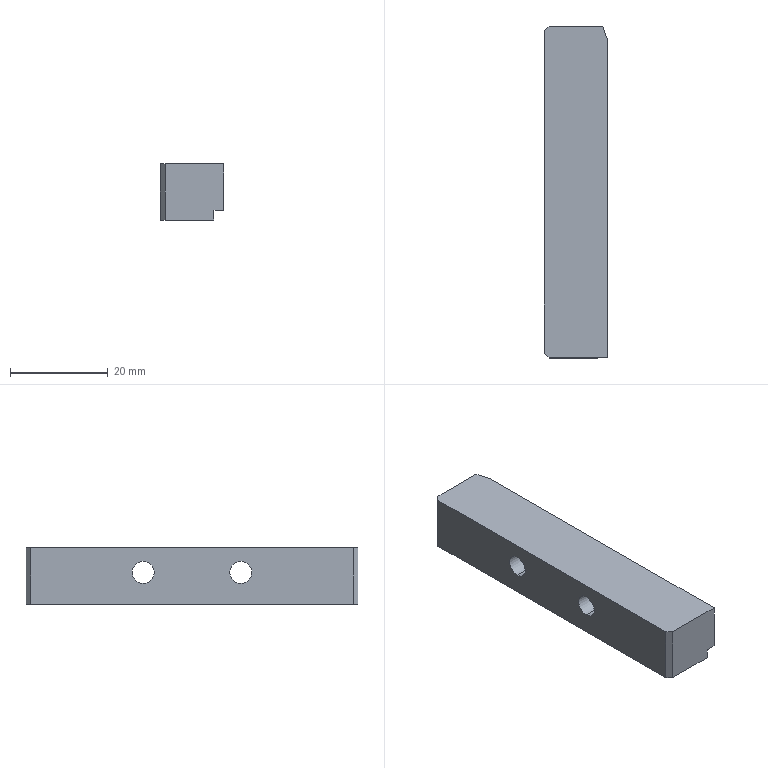Component | SolidWorks | 09HHHHH1-1 | 1 solid | 21 faces | box 13 x 68 x 11.5 mm | volume 9139 mm3 | plane 13 | cylinder 8 | commonest cylinder face diameters 8 x4 4.5 x4
build123d program:
from build123d import *

# Parameters (mm, degrees)
SKETCH1_W                                            = 13
SKETCH1_H                                            = 68
BOSS_EXTRUDE1_DEPTH                                  = 10
CUT_EXTRUDE1_DEPTH                                   = 652.1
HOLE_SIZE_ACCORDING_TO_THE_TYPE_OF_HEXAG_D           = 4.5
HOLE_SIZE_ACCORDING_TO_THE_TYPE_OF_HEXAG_CBORE_D     = 8
HOLE_SIZE_ACCORDING_TO_THE_TYPE_OF_HEXAG_CBORE_DEPTH = 4.6
CHAMFER1_SIZE                                        = 1
MOVE_FACE1_BY                                        = 1.5
SKETCH5_W                                            = 12.153
SKETCH5_H                                            = 73.603
CUT_EXTRUDE2_DEPTH                                   = 2


with BuildPart() as part:
    # Sketch1 → Boss-Extrude1 (new body)
    with BuildSketch(Plane.XY):
        with Locations((-555.859, -294)):
            Rectangle(SKETCH1_W, SKETCH1_H)
    extrude(amount=BOSS_EXTRUDE1_DEPTH)

    # Sketch2 → Cut-Extrude1 (cut, through all)
    with BuildSketch(Plane.XY.offset(10)):
        Polygon((-549.359, -260), (-550.359, -260), (-549.359, -263), align=None)
    extrude(amount=-CUT_EXTRUDE1_DEPTH, mode=Mode.SUBTRACT)

    # Hole Size according to the type of hexag (through all)
    with Locations(Plane(origin=(-549.359, 0, 0), x_dir=(0, 0, -1), z_dir=(1, 0, 0))):
        with Locations((-5, -284), (-5, -304)):
            CounterBoreHole(HOLE_SIZE_ACCORDING_TO_THE_TYPE_OF_HEXAG_D / 2, HOLE_SIZE_ACCORDING_TO_THE_TYPE_OF_HEXAG_CBORE_D / 2, HOLE_SIZE_ACCORDING_TO_THE_TYPE_OF_HEXAG_CBORE_DEPTH)

    # Chamfer1
    chamfer1_edges = [part.edges().sort_by_distance(p)[0] for p in [
        (-562.359, -260, 5),
        (-562.359, -328, 5),
    ]]
    chamfer(chamfer1_edges, length=CHAMFER1_SIZE)

    # Move Face1: a face moved outward by 1.5
    extrude(part.faces().sort_by_distance((-555.862, -294.056, 0))[0], amount=MOVE_FACE1_BY, dir=(0, 0, -1))

    # Sketch5 → Cut-Extrude2 (cut)
    with BuildSketch(Plane(origin=(-549.359, 0, 0), x_dir=(0, 0, -1), z_dir=(1, 0, 0))):
        with Locations((5.577, -293.944)):
            Rectangle(SKETCH5_W, SKETCH5_H)
    extrude(amount=-CUT_EXTRUDE2_DEPTH, mode=Mode.SUBTRACT)


solid = part.part

# Placed as in the assembly
solid = solid.moved(Location((-0.5807, 7.617, -1.156), (0, 0, 0)))
STEP:
#1=COLOUR_RGB('',0.7922,0.8196,0.9333);
#2=FILL_AREA_STYLE_COLOUR('',#1);
#3=FILL_AREA_STYLE('',(#2));
#4=SURFACE_STYLE_FILL_AREA(#3);
#5=SURFACE_SIDE_STYLE('',(#4));
#6=SURFACE_STYLE_USAGE(.BOTH.,#5);
#7=PRESENTATION_STYLE_ASSIGNMENT((#6));
#8=CARTESIAN_POINT('',(-21.832,-10.881,0.3088));
#9=VERTEX_POINT('',#8);
#10=CARTESIAN_POINT('',(-21.832,-10.881,-0.006151));
#11=VERTEX_POINT('',#10);
#12=CARTESIAN_POINT('',(-21.832,-10.881,0.1513));
#13=DIRECTION('',(1.,0.,0.));
#14=DIRECTION('',(0.,0.,-1.));
#15=AXIS2_PLACEMENT_3D('',#12,#13,#14);
#16=CIRCLE('',#15,0.1575);
#17=EDGE_CURVE('',#9,#11,#16,.T.);
#18=ORIENTED_EDGE('',*,*,#17,.F.);
#19=CARTESIAN_POINT('',(-21.651,-10.881,0.3088));
#20=VERTEX_POINT('',#19);
#21=CARTESIAN_POINT('',(-21.651,-10.881,0.3088));
#22=DIRECTION('',(1.,0.,0.));
#23=VECTOR('',#22,39.37);
#24=LINE('',#21,#23);
#25=EDGE_CURVE('',#9,#20,#24,.T.);
#26=ORIENTED_EDGE('',*,*,#25,.T.);
#27=CARTESIAN_POINT('',(-21.651,-10.881,-0.006151));
#28=VERTEX_POINT('',#27);
#29=CARTESIAN_POINT('',(-21.651,-10.881,0.1513));
#30=DIRECTION('',(1.,0.,0.));
#31=DIRECTION('',(0.,0.,-1.));
#32=AXIS2_PLACEMENT_3D('',#29,#30,#31);
#33=CIRCLE('',#32,0.1575);
#34=EDGE_CURVE('',#20,#28,#33,.T.);
#35=ORIENTED_EDGE('',*,*,#34,.T.);
#36=CARTESIAN_POINT('',(-21.651,-10.881,-0.006151));
#37=DIRECTION('',(1.,0.,0.));
#38=VECTOR('',#37,39.37);
#39=LINE('',#36,#38);
#40=EDGE_CURVE('',#11,#28,#39,.T.);
#41=ORIENTED_EDGE('',*,*,#40,.F.);
#42=EDGE_LOOP('',(#18,#26,#35,#41));
#43=FACE_OUTER_BOUND('',#42,.T.);
#44=CARTESIAN_POINT('',(-21.651,-10.881,0.1513));
#45=DIRECTION('',(1.,0.,0.));
#46=DIRECTION('',(0.,0.,-1.));
#47=AXIS2_PLACEMENT_3D('',#44,#45,#46);
#48=CYLINDRICAL_SURFACE('',#47,0.1575);
#49=ADVANCED_FACE('',(#43),#48,.F.);
#50=CARTESIAN_POINT('',(-22.163,-10.881,0.2399));
#51=VERTEX_POINT('',#50);
#52=CARTESIAN_POINT('',(-22.163,-10.881,0.06275));
#53=VERTEX_POINT('',#52);
#54=CARTESIAN_POINT('',(-22.163,-10.881,0.1513));
#55=DIRECTION('',(1.,0.,0.));
#56=DIRECTION('',(0.,0.,-1.));
#57=AXIS2_PLACEMENT_3D('',#54,#55,#56);
#58=CIRCLE('',#57,0.08858);
#59=EDGE_CURVE('',#51,#53,#58,.T.);
#60=ORIENTED_EDGE('',*,*,#59,.F.);
#61=CARTESIAN_POINT('',(-21.832,-10.881,0.2399));
#62=VERTEX_POINT('',#61);
#63=CARTESIAN_POINT('',(-21.651,-10.881,0.2399));
#64=DIRECTION('',(1.,0.,0.));
#65=VECTOR('',#64,39.37);
#66=LINE('',#63,#65);
#67=EDGE_CURVE('',#51,#62,#66,.T.);
#68=ORIENTED_EDGE('',*,*,#67,.T.);
#69=CARTESIAN_POINT('',(-21.832,-10.881,0.06275));
#70=VERTEX_POINT('',#69);
#71=CARTESIAN_POINT('',(-21.832,-10.881,0.1513));
#72=DIRECTION('',(1.,0.,0.));
#73=DIRECTION('',(0.,0.,-1.));
#74=AXIS2_PLACEMENT_3D('',#71,#72,#73);
#75=CIRCLE('',#74,0.08858);
#76=EDGE_CURVE('',#62,#70,#75,.T.);
#77=ORIENTED_EDGE('',*,*,#76,.T.);
#78=CARTESIAN_POINT('',(-21.651,-10.881,0.06275));
#79=DIRECTION('',(1.,0.,0.));
#80=VECTOR('',#79,39.37);
#81=LINE('',#78,#80);
#82=EDGE_CURVE('',#53,#70,#81,.T.);
#83=ORIENTED_EDGE('',*,*,#82,.F.);
#84=EDGE_LOOP('',(#60,#68,#77,#83));
#85=FACE_OUTER_BOUND('',#84,.T.);
#86=CARTESIAN_POINT('',(-21.651,-10.881,0.1513));
#87=DIRECTION('',(1.,0.,0.));
#88=DIRECTION('',(0.,0.,-1.));
#89=AXIS2_PLACEMENT_3D('',#86,#87,#88);
#90=CYLINDRICAL_SURFACE('',#89,0.08858);
#91=ADVANCED_FACE('',(#85),#90,.F.);
#92=CARTESIAN_POINT('',(-21.832,-11.669,0.3088));
#93=VERTEX_POINT('',#92);
#94=CARTESIAN_POINT('',(-21.832,-11.669,-0.006151));
#95=VERTEX_POINT('',#94);
#96=CARTESIAN_POINT('',(-21.832,-11.669,0.1513));
#97=DIRECTION('',(1.,0.,0.));
#98=DIRECTION('',(0.,0.,-1.));
#99=AXIS2_PLACEMENT_3D('',#96,#97,#98);
#100=CIRCLE('',#99,0.1575);
#101=EDGE_CURVE('',#93,#95,#100,.T.);
#102=ORIENTED_EDGE('',*,*,#101,.F.);
#103=CARTESIAN_POINT('',(-21.651,-11.669,0.3088));
#104=VERTEX_POINT('',#103);
#105=CARTESIAN_POINT('',(-21.651,-11.669,0.3088));
#106=DIRECTION('',(1.,0.,0.));
#107=VECTOR('',#106,39.37);
#108=LINE('',#105,#107);
#109=EDGE_CURVE('',#93,#104,#108,.T.);
#110=ORIENTED_EDGE('',*,*,#109,.T.);
#111=CARTESIAN_POINT('',(-21.651,-11.669,-0.006151));
#112=VERTEX_POINT('',#111);
#113=CARTESIAN_POINT('',(-21.651,-11.669,0.1513));
#114=DIRECTION('',(1.,0.,0.));
#115=DIRECTION('',(0.,0.,-1.));
#116=AXIS2_PLACEMENT_3D('',#113,#114,#115);
#117=CIRCLE('',#116,0.1575);
#118=EDGE_CURVE('',#104,#112,#117,.T.);
#119=ORIENTED_EDGE('',*,*,#118,.T.);
#120=CARTESIAN_POINT('',(-21.651,-11.669,-0.006151));
#121=DIRECTION('',(1.,0.,0.));
#122=VECTOR('',#121,39.37);
#123=LINE('',#120,#122);
#124=EDGE_CURVE('',#95,#112,#123,.T.);
#125=ORIENTED_EDGE('',*,*,#124,.F.);
#126=EDGE_LOOP('',(#102,#110,#119,#125));
#127=FACE_OUTER_BOUND('',#126,.T.);
#128=CARTESIAN_POINT('',(-21.651,-11.669,0.1513));
#129=DIRECTION('',(1.,0.,0.));
#130=DIRECTION('',(0.,0.,-1.));
#131=AXIS2_PLACEMENT_3D('',#128,#129,#130);
#132=CYLINDRICAL_SURFACE('',#131,0.1575);
#133=ADVANCED_FACE('',(#127),#132,.F.);
#134=CARTESIAN_POINT('',(-22.163,-11.669,0.2399));
#135=VERTEX_POINT('',#134);
#136=CARTESIAN_POINT('',(-22.163,-11.669,0.06275));
#137=VERTEX_POINT('',#136);
#138=CARTESIAN_POINT('',(-22.163,-11.669,0.1513));
#139=DIRECTION('',(1.,0.,0.));
#140=DIRECTION('',(0.,0.,-1.));
#141=AXIS2_PLACEMENT_3D('',#138,#139,#140);
#142=CIRCLE('',#141,0.08858);
#143=EDGE_CURVE('',#135,#137,#142,.T.);
#144=ORIENTED_EDGE('',*,*,#143,.F.);
#145=CARTESIAN_POINT('',(-21.832,-11.669,0.2399));
#146=VERTEX_POINT('',#145);
#147=CARTESIAN_POINT('',(-21.651,-11.669,0.2399));
#148=DIRECTION('',(1.,0.,0.));
#149=VECTOR('',#148,39.37);
#150=LINE('',#147,#149);
#151=EDGE_CURVE('',#135,#146,#150,.T.);
#152=ORIENTED_EDGE('',*,*,#151,.T.);
#153=CARTESIAN_POINT('',(-21.832,-11.669,0.06275));
#154=VERTEX_POINT('',#153);
#155=CARTESIAN_POINT('',(-21.832,-11.669,0.1513));
#156=DIRECTION('',(1.,0.,0.));
#157=DIRECTION('',(0.,0.,-1.));
#158=AXIS2_PLACEMENT_3D('',#155,#156,#157);
#159=CIRCLE('',#158,0.08858);
#160=EDGE_CURVE('',#146,#154,#159,.T.);
#161=ORIENTED_EDGE('',*,*,#160,.T.);
#162=CARTESIAN_POINT('',(-21.651,-11.669,0.06275));
#163=DIRECTION('',(1.,0.,0.));
#164=VECTOR('',#163,39.37);
#165=LINE('',#162,#164);
#166=EDGE_CURVE('',#137,#154,#165,.T.);
#167=ORIENTED_EDGE('',*,*,#166,.F.);
#168=EDGE_LOOP('',(#144,#152,#161,#167));
#169=FACE_OUTER_BOUND('',#168,.T.);
#170=CARTESIAN_POINT('',(-21.651,-11.669,0.1513));
#171=DIRECTION('',(1.,0.,0.));
#172=DIRECTION('',(0.,0.,-1.));
#173=AXIS2_PLACEMENT_3D('',#170,#171,#172);
#174=CYLINDRICAL_SURFACE('',#173,0.08858);
#175=ADVANCED_FACE('',(#169),#174,.F.);
#176=CARTESIAN_POINT('',(-21.73,-9.936,-0.1046));
#177=VERTEX_POINT('',#176);
#178=CARTESIAN_POINT('',(-22.124,-9.936,-0.1046));
#179=VERTEX_POINT('',#178);
#180=CARTESIAN_POINT('',(-0.02286,-9.936,-0.1046));
#181=DIRECTION('',(-1.,0.,0.));
#182=VECTOR('',#181,39.37);
#183=LINE('',#180,#182);
#184=EDGE_CURVE('',#177,#179,#183,.T.);
#185=ORIENTED_EDGE('',*,*,#184,.F.);
#186=CARTESIAN_POINT('',(-21.73,-12.614,-0.1046));
#187=VERTEX_POINT('',#186);
#188=CARTESIAN_POINT('',(-21.73,0.2999,-0.1046));
#189=DIRECTION('',(0.,-1.,0.));
#190=VECTOR('',#189,39.37);
#191=LINE('',#188,#190);
#192=EDGE_CURVE('',#177,#187,#191,.T.);
#193=ORIENTED_EDGE('',*,*,#192,.T.);
#194=CARTESIAN_POINT('',(-22.124,-12.614,-0.1046));
#195=VERTEX_POINT('',#194);
#196=CARTESIAN_POINT('',(-0.02286,-12.614,-0.1046));
#197=DIRECTION('',(1.,0.,0.));
#198=VECTOR('',#197,39.37);
#199=LINE('',#196,#198);
#200=EDGE_CURVE('',#195,#187,#199,.T.);
#201=ORIENTED_EDGE('',*,*,#200,.F.);
#202=CARTESIAN_POINT('',(-22.163,-12.574,-0.1046));
#203=VERTEX_POINT('',#202);
#204=CARTESIAN_POINT('',(-17.53,-17.207,-0.1046));
#205=DIRECTION('',(-0.7071,0.7071,0.));
#206=VECTOR('',#205,39.37);
#207=LINE('',#204,#206);
#208=EDGE_CURVE('',#195,#203,#207,.T.);
#209=ORIENTED_EDGE('',*,*,#208,.T.);
#210=CARTESIAN_POINT('',(-22.163,-9.976,-0.1046));
#211=VERTEX_POINT('',#210);
#212=CARTESIAN_POINT('',(-22.163,0.2999,-0.1046));
#213=DIRECTION('',(0.,-1.,0.));
#214=VECTOR('',#213,39.37);
#215=LINE('',#212,#214);
#216=EDGE_CURVE('',#211,#203,#215,.T.);
#217=ORIENTED_EDGE('',*,*,#216,.F.);
#218=CARTESIAN_POINT('',(-5.955,6.232,-0.1046));
#219=DIRECTION('',(0.7071,0.7071,0.));
#220=VECTOR('',#219,39.37);
#221=LINE('',#218,#220);
#222=EDGE_CURVE('',#211,#179,#221,.T.);
#223=ORIENTED_EDGE('',*,*,#222,.T.);
#224=EDGE_LOOP('',(#185,#193,#201,#209,#217,#223));
#225=FACE_OUTER_BOUND('',#224,.T.);
#226=CARTESIAN_POINT('',(-0.02286,0.2999,-0.1046));
#227=DIRECTION('',(0.,0.,-1.));
#228=DIRECTION('',(-1.,0.,0.));
#229=AXIS2_PLACEMENT_3D('',#226,#227,#228);
#230=PLANE('',#229);
#231=ADVANCED_FACE('',(#225),#230,.T.);
#232=CARTESIAN_POINT('',(-21.651,-11.669,0.1513));
#233=DIRECTION('',(1.,0.,0.));
#234=DIRECTION('',(0.,0.,-1.));
#235=AXIS2_PLACEMENT_3D('',#232,#233,#234);
#236=CIRCLE('',#235,0.1575);
#237=EDGE_CURVE('',#112,#104,#236,.T.);
#238=ORIENTED_EDGE('',*,*,#237,.F.);
#239=ORIENTED_EDGE('',*,*,#118,.F.);
#240=EDGE_LOOP('',(#238,#239));
#241=FACE_BOUND('',#240,.T.);
#242=CARTESIAN_POINT('',(-21.651,-12.614,0.3482));
#243=VERTEX_POINT('',#242);
#244=CARTESIAN_POINT('',(-21.651,-12.614,-0.02584));
#245=VERTEX_POINT('',#244);
#246=CARTESIAN_POINT('',(-21.651,-12.614,0.3482));
#247=DIRECTION('',(0.,0.,-1.));
#248=VECTOR('',#247,39.37);
#249=LINE('',#246,#248);
#250=EDGE_CURVE('',#243,#245,#249,.T.);
#251=ORIENTED_EDGE('',*,*,#250,.T.);
#252=CARTESIAN_POINT('',(-21.651,-10.054,-0.02584));
#253=VERTEX_POINT('',#252);
#254=CARTESIAN_POINT('',(-21.651,-9.824,-0.02584));
#255=DIRECTION('',(0.,-1.,-0.));
#256=VECTOR('',#255,39.37);
#257=LINE('',#254,#256);
#258=EDGE_CURVE('',#253,#245,#257,.T.);
#259=ORIENTED_EDGE('',*,*,#258,.F.);
#260=CARTESIAN_POINT('',(-21.651,-10.054,0.3482));
#261=VERTEX_POINT('',#260);
#262=CARTESIAN_POINT('',(-21.651,-10.054,-0.04552));
#263=DIRECTION('',(0.,0.,1.));
#264=VECTOR('',#263,39.37);
#265=LINE('',#262,#264);
#266=EDGE_CURVE('',#253,#261,#265,.T.);
#267=ORIENTED_EDGE('',*,*,#266,.T.);
#268=CARTESIAN_POINT('',(-21.651,-12.614,0.3482));
#269=DIRECTION('',(0.,1.,0.));
#270=VECTOR('',#269,39.37);
#271=LINE('',#268,#270);
#272=EDGE_CURVE('',#243,#261,#271,.T.);
#273=ORIENTED_EDGE('',*,*,#272,.F.);
#274=EDGE_LOOP('',(#251,#259,#267,#273));
#275=FACE_OUTER_BOUND('',#274,.T.);
#276=CARTESIAN_POINT('',(-21.651,-10.881,0.1513));
#277=DIRECTION('',(1.,0.,0.));
#278=DIRECTION('',(0.,0.,-1.));
#279=AXIS2_PLACEMENT_3D('',#276,#277,#278);
#280=CIRCLE('',#279,0.1575);
#281=EDGE_CURVE('',#28,#20,#280,.T.);
#282=ORIENTED_EDGE('',*,*,#281,.F.);
#283=ORIENTED_EDGE('',*,*,#34,.F.);
#284=EDGE_LOOP('',(#282,#283));
#285=FACE_BOUND('',#284,.T.);
#286=CARTESIAN_POINT('',(-21.651,-12.614,0.3482));
#287=DIRECTION('',(-1.,0.,0.));
#288=DIRECTION('',(0.,0.,1.));
#289=AXIS2_PLACEMENT_3D('',#286,#287,#288);
#290=PLANE('',#289);
#291=ADVANCED_FACE('',(#241,#275,#285),#290,.F.);
#292=CARTESIAN_POINT('',(-22.163,-10.881,0.1513));
#293=DIRECTION('',(1.,0.,0.));
#294=DIRECTION('',(0.,0.,-1.));
#295=AXIS2_PLACEMENT_3D('',#292,#293,#294);
#296=CIRCLE('',#295,0.08858);
#297=EDGE_CURVE('',#53,#51,#296,.T.);
#298=ORIENTED_EDGE('',*,*,#297,.T.);
#299=ORIENTED_EDGE('',*,*,#59,.T.);
#300=EDGE_LOOP('',(#298,#299));
#301=FACE_BOUND('',#300,.T.);
#302=CARTESIAN_POINT('',(-22.163,-11.669,0.1513));
#303=DIRECTION('',(1.,0.,0.));
#304=DIRECTION('',(0.,0.,-1.));
#305=AXIS2_PLACEMENT_3D('',#302,#303,#304);
#306=CIRCLE('',#305,0.08858);
#307=EDGE_CURVE('',#137,#135,#306,.T.);
#308=ORIENTED_EDGE('',*,*,#307,.T.);
#309=ORIENTED_EDGE('',*,*,#143,.T.);
#310=EDGE_LOOP('',(#308,#309));
#311=FACE_BOUND('',#310,.T.);
#312=ORIENTED_EDGE('',*,*,#216,.T.);
#313=CARTESIAN_POINT('',(-22.163,-12.574,0.3482));
#314=VERTEX_POINT('',#313);
#315=CARTESIAN_POINT('',(-22.163,-12.574,0.3482));
#316=DIRECTION('',(0.,0.,1.));
#317=VECTOR('',#316,39.37);
#318=LINE('',#315,#317);
#319=EDGE_CURVE('',#203,#314,#318,.T.);
#320=ORIENTED_EDGE('',*,*,#319,.T.);
#321=CARTESIAN_POINT('',(-22.163,-9.976,0.3482));
#322=VERTEX_POINT('',#321);
#323=CARTESIAN_POINT('',(-22.163,-12.614,0.3482));
#324=DIRECTION('',(0.,-1.,0.));
#325=VECTOR('',#324,39.37);
#326=LINE('',#323,#325);
#327=EDGE_CURVE('',#322,#314,#326,.T.);
#328=ORIENTED_EDGE('',*,*,#327,.F.);
#329=CARTESIAN_POINT('',(-22.163,-9.976,0.3482));
#330=DIRECTION('',(0.,0.,-1.));
#331=VECTOR('',#330,39.37);
#332=LINE('',#329,#331);
#333=EDGE_CURVE('',#322,#211,#332,.T.);
#334=ORIENTED_EDGE('',*,*,#333,.T.);
#335=EDGE_LOOP('',(#312,#320,#328,#334));
#336=FACE_OUTER_BOUND('',#335,.T.);
#337=CARTESIAN_POINT('',(-22.163,-12.614,0.3482));
#338=DIRECTION('',(1.,0.,0.));
#339=DIRECTION('',(0.,0.,-1.));
#340=AXIS2_PLACEMENT_3D('',#337,#338,#339);
#341=PLANE('',#340);
#342=ADVANCED_FACE('',(#301,#311,#336),#341,.F.);
#343=CARTESIAN_POINT('',(-21.73,-12.614,-0.02584));
#344=VERTEX_POINT('',#343);
#345=CARTESIAN_POINT('',(-21.73,-12.614,0.3482));
#346=DIRECTION('',(0.,0.,-1.));
#347=VECTOR('',#346,39.37);
#348=LINE('',#345,#347);
#349=EDGE_CURVE('',#344,#187,#348,.T.);
#350=ORIENTED_EDGE('',*,*,#349,.F.);
#351=CARTESIAN_POINT('',(-22.163,-12.614,-0.02584));
#352=DIRECTION('',(1.,0.,0.));
#353=VECTOR('',#352,39.37);
#354=LINE('',#351,#353);
#355=EDGE_CURVE('',#344,#245,#354,.T.);
#356=ORIENTED_EDGE('',*,*,#355,.T.);
#357=ORIENTED_EDGE('',*,*,#250,.F.);
#358=CARTESIAN_POINT('',(-22.124,-12.614,0.3482));
#359=VERTEX_POINT('',#358);
#360=CARTESIAN_POINT('',(-22.163,-12.614,0.3482));
#361=DIRECTION('',(1.,0.,0.));
#362=VECTOR('',#361,39.37);
#363=LINE('',#360,#362);
#364=EDGE_CURVE('',#359,#243,#363,.T.);
#365=ORIENTED_EDGE('',*,*,#364,.F.);
#366=CARTESIAN_POINT('',(-22.124,-12.614,0.3482));
#367=DIRECTION('',(0.,0.,-1.));
#368=VECTOR('',#367,39.37);
#369=LINE('',#366,#368);
#370=EDGE_CURVE('',#359,#195,#369,.T.);
#371=ORIENTED_EDGE('',*,*,#370,.T.);
#372=ORIENTED_EDGE('',*,*,#200,.T.);
#373=EDGE_LOOP('',(#350,#356,#357,#365,#371,#372));
#374=FACE_OUTER_BOUND('',#373,.T.);
#375=CARTESIAN_POINT('',(-22.163,-12.614,0.3482));
#376=DIRECTION('',(0.,1.,0.));
#377=DIRECTION('',(0.,0.,1.));
#378=AXIS2_PLACEMENT_3D('',#375,#376,#377);
#379=PLANE('',#378);
#380=ADVANCED_FACE('',(#374),#379,.F.);
#381=CARTESIAN_POINT('',(-21.691,-9.936,-0.02584));
#382=VERTEX_POINT('',#381);
#383=CARTESIAN_POINT('',(-21.691,-9.936,0.3482));
#384=VERTEX_POINT('',#383);
#385=CARTESIAN_POINT('',(-21.691,-9.936,-0.04552));
#386=DIRECTION('',(0.,0.,1.));
#387=VECTOR('',#386,39.37);
#388=LINE('',#385,#387);
#389=EDGE_CURVE('',#382,#384,#388,.T.);
#390=ORIENTED_EDGE('',*,*,#389,.F.);
#391=CARTESIAN_POINT('',(-21.73,-9.936,-0.02584));
#392=VERTEX_POINT('',#391);
#393=CARTESIAN_POINT('',(-22.163,-9.936,-0.02584));
#394=DIRECTION('',(-1.,0.,0.));
#395=VECTOR('',#394,39.37);
#396=LINE('',#393,#395);
#397=EDGE_CURVE('',#382,#392,#396,.T.);
#398=ORIENTED_EDGE('',*,*,#397,.T.);
#399=CARTESIAN_POINT('',(-21.73,-9.936,0.3482));
#400=DIRECTION('',(0.,0.,1.));
#401=VECTOR('',#400,39.37);
#402=LINE('',#399,#401);
#403=EDGE_CURVE('',#177,#392,#402,.T.);
#404=ORIENTED_EDGE('',*,*,#403,.F.);
#405=ORIENTED_EDGE('',*,*,#184,.T.);
#406=CARTESIAN_POINT('',(-22.124,-9.936,0.3482));
#407=VERTEX_POINT('',#406);
#408=CARTESIAN_POINT('',(-22.124,-9.936,0.3482));
#409=DIRECTION('',(0.,0.,1.));
#410=VECTOR('',#409,39.37);
#411=LINE('',#408,#410);
#412=EDGE_CURVE('',#179,#407,#411,.T.);
#413=ORIENTED_EDGE('',*,*,#412,.T.);
#414=CARTESIAN_POINT('',(-22.163,-9.936,0.3482));
#415=DIRECTION('',(-1.,0.,0.));
#416=VECTOR('',#415,39.37);
#417=LINE('',#414,#416);
#418=EDGE_CURVE('',#384,#407,#417,.T.);
#419=ORIENTED_EDGE('',*,*,#418,.F.);
#420=EDGE_LOOP('',(#390,#398,#404,#405,#413,#419));
#421=FACE_OUTER_BOUND('',#420,.T.);
#422=CARTESIAN_POINT('',(-22.163,-9.936,0.3482));
#423=DIRECTION('',(0.,-1.,0.));
#424=DIRECTION('',(0.,0.,-1.));
#425=AXIS2_PLACEMENT_3D('',#422,#423,#424);
#426=PLANE('',#425);
#427=ADVANCED_FACE('',(#421),#426,.F.);
#428=ORIENTED_EDGE('',*,*,#327,.T.);
#429=CARTESIAN_POINT('',(-22.124,-12.614,0.3482));
#430=DIRECTION('',(0.7071,-0.7071,0.));
#431=VECTOR('',#430,39.37);
#432=LINE('',#429,#431);
#433=EDGE_CURVE('',#314,#359,#432,.T.);
#434=ORIENTED_EDGE('',*,*,#433,.T.);
#435=ORIENTED_EDGE('',*,*,#364,.T.);
#436=ORIENTED_EDGE('',*,*,#272,.T.);
#437=CARTESIAN_POINT('',(-21.691,-9.936,0.3482));
#438=DIRECTION('',(0.3162,-0.9487,0.));
#439=VECTOR('',#438,39.37);
#440=LINE('',#437,#439);
#441=EDGE_CURVE('',#384,#261,#440,.T.);
#442=ORIENTED_EDGE('',*,*,#441,.F.);
#443=ORIENTED_EDGE('',*,*,#418,.T.);
#444=CARTESIAN_POINT('',(-22.163,-9.976,0.3482));
#445=DIRECTION('',(-0.7071,-0.7071,0.));
#446=VECTOR('',#445,39.37);
#447=LINE('',#444,#446);
#448=EDGE_CURVE('',#407,#322,#447,.T.);
#449=ORIENTED_EDGE('',*,*,#448,.T.);
#450=EDGE_LOOP('',(#428,#434,#435,#436,#442,#443,#449));
#451=FACE_OUTER_BOUND('',#450,.T.);
#452=CARTESIAN_POINT('',(-0.02286,0.2999,0.3482));
#453=DIRECTION('',(0.,0.,-1.));
#454=DIRECTION('',(-1.,0.,0.));
#455=AXIS2_PLACEMENT_3D('',#452,#453,#454);
#456=PLANE('',#455);
#457=ADVANCED_FACE('',(#451),#456,.F.);
#458=ORIENTED_EDGE('',*,*,#266,.F.);
#459=CARTESIAN_POINT('',(-21.691,-9.936,-0.02584));
#460=DIRECTION('',(-0.3162,0.9487,0.));
#461=VECTOR('',#460,39.37);
#462=LINE('',#459,#461);
#463=EDGE_CURVE('',#253,#382,#462,.T.);
#464=ORIENTED_EDGE('',*,*,#463,.T.);
#465=ORIENTED_EDGE('',*,*,#389,.T.);
#466=ORIENTED_EDGE('',*,*,#441,.T.);
#467=EDGE_LOOP('',(#458,#464,#465,#466));
#468=FACE_OUTER_BOUND('',#467,.T.);
#469=CARTESIAN_POINT('',(-21.691,-9.936,-0.04552));
#470=DIRECTION('',(-0.9487,-0.3162,0.));
#471=DIRECTION('',(0.3162,-0.9487,0.));
#472=AXIS2_PLACEMENT_3D('',#469,#470,#471);
#473=PLANE('',#472);
#474=ADVANCED_FACE('',(#468),#473,.F.);
#475=ORIENTED_EDGE('',*,*,#151,.F.);
#476=ORIENTED_EDGE('',*,*,#307,.F.);
#477=ORIENTED_EDGE('',*,*,#166,.T.);
#478=CARTESIAN_POINT('',(-21.832,-11.669,0.1513));
#479=DIRECTION('',(1.,0.,0.));
#480=DIRECTION('',(0.,0.,-1.));
#481=AXIS2_PLACEMENT_3D('',#478,#479,#480);
#482=CIRCLE('',#481,0.08858);
#483=EDGE_CURVE('',#154,#146,#482,.T.);
#484=ORIENTED_EDGE('',*,*,#483,.T.);
#485=EDGE_LOOP('',(#475,#476,#477,#484));
#486=FACE_OUTER_BOUND('',#485,.T.);
#487=CARTESIAN_POINT('',(-21.651,-11.669,0.1513));
#488=DIRECTION('',(1.,0.,0.));
#489=DIRECTION('',(0.,0.,-1.));
#490=AXIS2_PLACEMENT_3D('',#487,#488,#489);
#491=CYLINDRICAL_SURFACE('',#490,0.08858);
#492=ADVANCED_FACE('',(#486),#491,.F.);
#493=ORIENTED_EDGE('',*,*,#483,.F.);
#494=ORIENTED_EDGE('',*,*,#160,.F.);
#495=EDGE_LOOP('',(#493,#494));
#496=FACE_BOUND('',#495,.T.);
#497=CARTESIAN_POINT('',(-21.832,-11.669,0.1513));
#498=DIRECTION('',(1.,0.,0.));
#499=DIRECTION('',(0.,0.,-1.));
#500=AXIS2_PLACEMENT_3D('',#497,#498,#499);
#501=CIRCLE('',#500,0.1575);
#502=EDGE_CURVE('',#95,#93,#501,.T.);
#503=ORIENTED_EDGE('',*,*,#502,.T.);
#504=ORIENTED_EDGE('',*,*,#101,.T.);
#505=EDGE_LOOP('',(#503,#504));
#506=FACE_OUTER_BOUND('',#505,.T.);
#507=CARTESIAN_POINT('',(-21.832,-11.58,0.1513));
#508=DIRECTION('',(-1.,0.,0.));
#509=DIRECTION('',(0.,0.,1.));
#510=AXIS2_PLACEMENT_3D('',#507,#508,#509);
#511=PLANE('',#510);
#512=ADVANCED_FACE('',(#496,#506),#511,.F.);
#513=ORIENTED_EDGE('',*,*,#109,.F.);
#514=ORIENTED_EDGE('',*,*,#502,.F.);
#515=ORIENTED_EDGE('',*,*,#124,.T.);
#516=ORIENTED_EDGE('',*,*,#237,.T.);
#517=EDGE_LOOP('',(#513,#514,#515,#516));
#518=FACE_OUTER_BOUND('',#517,.T.);
#519=CARTESIAN_POINT('',(-21.651,-11.669,0.1513));
#520=DIRECTION('',(1.,0.,0.));
#521=DIRECTION('',(0.,0.,-1.));
#522=AXIS2_PLACEMENT_3D('',#519,#520,#521);
#523=CYLINDRICAL_SURFACE('',#522,0.1575);
#524=ADVANCED_FACE('',(#518),#523,.F.);
#525=ORIENTED_EDGE('',*,*,#67,.F.);
#526=ORIENTED_EDGE('',*,*,#297,.F.);
#527=ORIENTED_EDGE('',*,*,#82,.T.);
#528=CARTESIAN_POINT('',(-21.832,-10.881,0.1513));
#529=DIRECTION('',(1.,0.,0.));
#530=DIRECTION('',(0.,0.,-1.));
#531=AXIS2_PLACEMENT_3D('',#528,#529,#530);
#532=CIRCLE('',#531,0.08858);
#533=EDGE_CURVE('',#70,#62,#532,.T.);
#534=ORIENTED_EDGE('',*,*,#533,.T.);
#535=EDGE_LOOP('',(#525,#526,#527,#534));
#536=FACE_OUTER_BOUND('',#535,.T.);
#537=CARTESIAN_POINT('',(-21.651,-10.881,0.1513));
#538=DIRECTION('',(1.,0.,0.));
#539=DIRECTION('',(0.,0.,-1.));
#540=AXIS2_PLACEMENT_3D('',#537,#538,#539);
#541=CYLINDRICAL_SURFACE('',#540,0.08858);
#542=ADVANCED_FACE('',(#536),#541,.F.);
#543=ORIENTED_EDGE('',*,*,#533,.F.);
#544=ORIENTED_EDGE('',*,*,#76,.F.);
#545=EDGE_LOOP('',(#543,#544));
#546=FACE_BOUND('',#545,.T.);
#547=CARTESIAN_POINT('',(-21.832,-10.881,0.1513));
#548=DIRECTION('',(1.,0.,0.));
#549=DIRECTION('',(0.,0.,-1.));
#550=AXIS2_PLACEMENT_3D('',#547,#548,#549);
#551=CIRCLE('',#550,0.1575);
#552=EDGE_CURVE('',#11,#9,#551,.T.);
#553=ORIENTED_EDGE('',*,*,#552,.T.);
#554=ORIENTED_EDGE('',*,*,#17,.T.);
#555=EDGE_LOOP('',(#553,#554));
#556=FACE_OUTER_BOUND('',#555,.T.);
#557=CARTESIAN_POINT('',(-21.832,-10.793,0.1513));
#558=DIRECTION('',(-1.,0.,0.));
#559=DIRECTION('',(0.,0.,1.));
#560=AXIS2_PLACEMENT_3D('',#557,#558,#559);
#561=PLANE('',#560);
#562=ADVANCED_FACE('',(#546,#556),#561,.F.);
#563=ORIENTED_EDGE('',*,*,#25,.F.);
#564=ORIENTED_EDGE('',*,*,#552,.F.);
#565=ORIENTED_EDGE('',*,*,#40,.T.);
#566=ORIENTED_EDGE('',*,*,#281,.T.);
#567=EDGE_LOOP('',(#563,#564,#565,#566));
#568=FACE_OUTER_BOUND('',#567,.T.);
#569=CARTESIAN_POINT('',(-21.651,-10.881,0.1513));
#570=DIRECTION('',(1.,0.,0.));
#571=DIRECTION('',(0.,0.,-1.));
#572=AXIS2_PLACEMENT_3D('',#569,#570,#571);
#573=CYLINDRICAL_SURFACE('',#572,0.1575);
#574=ADVANCED_FACE('',(#568),#573,.F.);
#575=ORIENTED_EDGE('',*,*,#433,.F.);
#576=ORIENTED_EDGE('',*,*,#319,.F.);
#577=ORIENTED_EDGE('',*,*,#208,.F.);
#578=ORIENTED_EDGE('',*,*,#370,.F.);
#579=EDGE_LOOP('',(#575,#576,#577,#578));
#580=FACE_OUTER_BOUND('',#579,.T.);
#581=CARTESIAN_POINT('',(-22.124,-12.614,0.3482));
#582=DIRECTION('',(0.7071,0.7071,0.));
#583=DIRECTION('',(0.,0.,-1.));
#584=AXIS2_PLACEMENT_3D('',#581,#582,#583);
#585=PLANE('',#584);
#586=ADVANCED_FACE('',(#580),#585,.F.);
#587=ORIENTED_EDGE('',*,*,#448,.F.);
#588=ORIENTED_EDGE('',*,*,#412,.F.);
#589=ORIENTED_EDGE('',*,*,#222,.F.);
#590=ORIENTED_EDGE('',*,*,#333,.F.);
#591=EDGE_LOOP('',(#587,#588,#589,#590));
#592=FACE_OUTER_BOUND('',#591,.T.);
#593=CARTESIAN_POINT('',(-22.163,-9.976,0.3482));
#594=DIRECTION('',(0.7071,-0.7071,0.));
#595=DIRECTION('',(0.,0.,-1.));
#596=AXIS2_PLACEMENT_3D('',#593,#594,#595);
#597=PLANE('',#596);
#598=ADVANCED_FACE('',(#592),#597,.F.);
#599=ORIENTED_EDGE('',*,*,#349,.T.);
#600=ORIENTED_EDGE('',*,*,#192,.F.);
#601=ORIENTED_EDGE('',*,*,#403,.T.);
#602=CARTESIAN_POINT('',(-21.73,-9.824,-0.02584));
#603=DIRECTION('',(0.,-1.,-0.));
#604=VECTOR('',#603,39.37);
#605=LINE('',#602,#604);
#606=EDGE_CURVE('',#392,#344,#605,.T.);
#607=ORIENTED_EDGE('',*,*,#606,.T.);
#608=EDGE_LOOP('',(#599,#600,#601,#607));
#609=FACE_OUTER_BOUND('',#608,.T.);
#610=CARTESIAN_POINT('',(-21.73,0.2999,-0.04552));
#611=DIRECTION('',(1.,0.,0.));
#612=DIRECTION('',(0.,0.,-1.));
#613=AXIS2_PLACEMENT_3D('',#610,#611,#612);
#614=PLANE('',#613);
#615=ADVANCED_FACE('',(#609),#614,.T.);
#616=ORIENTED_EDGE('',*,*,#606,.F.);
#617=ORIENTED_EDGE('',*,*,#397,.F.);
#618=ORIENTED_EDGE('',*,*,#463,.F.);
#619=ORIENTED_EDGE('',*,*,#258,.T.);
#620=ORIENTED_EDGE('',*,*,#355,.F.);
#621=EDGE_LOOP('',(#616,#617,#618,#619,#620));
#622=FACE_OUTER_BOUND('',#621,.T.);
#623=CARTESIAN_POINT('',(-21.73,-9.824,-0.02584));
#624=DIRECTION('',(0.,-0.,1.));
#625=DIRECTION('',(0.,-1.,-0.));
#626=AXIS2_PLACEMENT_3D('',#623,#624,#625);
#627=PLANE('',#626);
#628=ADVANCED_FACE('',(#622),#627,.F.);
#629=CLOSED_SHELL('',(#49,#91,#133,#175,#231,#291,#342,#380,#427,#457,#474,#492,#512,#524,#542,#562,#574,#586,#598,#615,#628));
#630=MANIFOLD_SOLID_BREP('',#629);
#631=STYLED_ITEM('',(#7),#630);
#632=PRESENTATION_LAYER_ASSIGNMENT('','',(#631));
#633=(LENGTH_UNIT()NAMED_UNIT(*)SI_UNIT($,.METRE.));
#634=LENGTH_MEASURE_WITH_UNIT(LENGTH_MEASURE(0.0254),#633);
#635=DIMENSIONAL_EXPONENTS(1.,0.,0.,0.,0.,0.,0.);
#636=(CONVERSION_BASED_UNIT('',#634)LENGTH_UNIT()NAMED_UNIT(#635));
#637=UNCERTAINTY_MEASURE_WITH_UNIT(LENGTH_MEASURE(0.00001),#636,'','');
#638=(NAMED_UNIT(*)PLANE_ANGLE_UNIT()SI_UNIT($,.RADIAN.));
#639=(NAMED_UNIT(*)SI_UNIT($,.STERADIAN.)SOLID_ANGLE_UNIT());
#640=(GEOMETRIC_REPRESENTATION_CONTEXT(3)GLOBAL_UNCERTAINTY_ASSIGNED_CONTEXT((#637))GLOBAL_UNIT_ASSIGNED_CONTEXT((#636,#638,#639))REPRESENTATION_CONTEXT('',''));
#641=MECHANICAL_DESIGN_GEOMETRIC_PRESENTATION_REPRESENTATION('',(#631),#640);
#642=CARTESIAN_POINT('',(0.,0.,0.));
#643=DIRECTION('',(0.,0.,1.));
#644=DIRECTION('',(1.,0.,0.));
#645=AXIS2_PLACEMENT_3D('',#642,#643,#644);
#646=(LENGTH_UNIT()NAMED_UNIT(*)SI_UNIT($,.METRE.));
#647=LENGTH_MEASURE_WITH_UNIT(LENGTH_MEASURE(0.0254),#646);
#648=DIMENSIONAL_EXPONENTS(1.,0.,0.,0.,0.,0.,0.);
#649=(CONVERSION_BASED_UNIT('',#647)LENGTH_UNIT()NAMED_UNIT(#648));
#650=UNCERTAINTY_MEASURE_WITH_UNIT(LENGTH_MEASURE(0.00001),#649,'','');
#651=(NAMED_UNIT(*)PLANE_ANGLE_UNIT()SI_UNIT($,.RADIAN.));
#652=(NAMED_UNIT(*)SI_UNIT($,.STERADIAN.)SOLID_ANGLE_UNIT());
#653=(GEOMETRIC_REPRESENTATION_CONTEXT(3)GLOBAL_UNCERTAINTY_ASSIGNED_CONTEXT((#650))GLOBAL_UNIT_ASSIGNED_CONTEXT((#649,#651,#652))REPRESENTATION_CONTEXT('',''));
#654=ADVANCED_BREP_SHAPE_REPRESENTATION('',(#630,#645),#653);